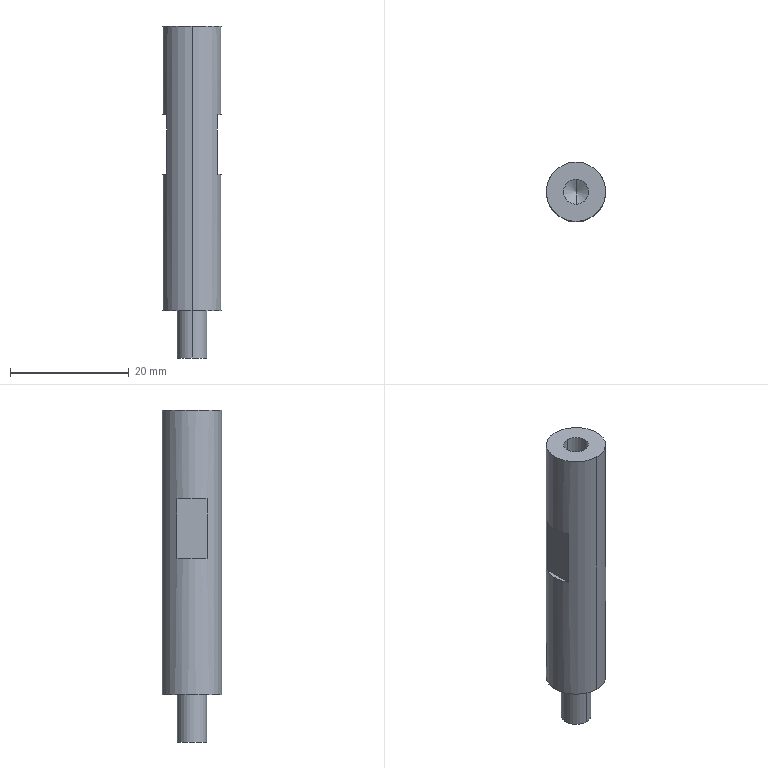Component | SolidWorks | YS01-059CylinderExtensionRod-2 | 1 solid | 17 faces | box 10 x 10 x 56 mm | volume 3701 mm3 | plane 9 | cylinder 6 | cone 2 | commonest cylinder face diameters 5 x2 4.2 x2 10 x2
build123d program:
from build123d import *

# Parameters (mm, degrees)
SKETCH1_R             = 5
BOSS_EXTRUDE1_DEPTH   = 48
M5_TAPPED_HOLE1_D     = 4.2
M5_TAPPED_HOLE1_DEPTH = 12.4
M5_TAPPED_HOLE1_TIP   = 1.262
SKETCH4_R             = 2.5
BOSS_EXTRUDE2_DEPTH   = 8
SKETCH5_W             = 15.912
SKETCH5_H             = 5.844
SKETCH5_H_2           = 6.454
CUT_EXTRUDE1_DEPTH    = 10


with BuildPart() as part:
    # Sketch1 → Boss-Extrude1 (new body)
    with BuildSketch(Plane.XY):
        Circle(SKETCH1_R)
    extrude(amount=BOSS_EXTRUDE1_DEPTH)

    # M5 Tapped Hole1
    with Locations(Plane.XY.offset(48)):
        with Locations((0, 0)):
            Hole(M5_TAPPED_HOLE1_D / 2, depth=M5_TAPPED_HOLE1_DEPTH)
            with Locations((0, 0, -(M5_TAPPED_HOLE1_DEPTH + M5_TAPPED_HOLE1_TIP / 2))):  # 118° drill point
                Cone(0, M5_TAPPED_HOLE1_D / 2, M5_TAPPED_HOLE1_TIP, mode=Mode.SUBTRACT)

    # Sketch4 → Boss-Extrude2 (add)
    with BuildSketch(Plane(origin=(0, 0, 0), x_dir=(-1, 0, 0), z_dir=(0, 0, -1))):
        with Locations(Location((0, 0, 0), (0, 0, 180))):
            Circle(SKETCH4_R)
    extrude(amount=BOSS_EXTRUDE2_DEPTH)

    # Sketch5 → Cut-Extrude1 (cut)
    with BuildSketch(Plane.XY.offset(33)):
        with Locations((1.405, 7.222)):
            Rectangle(SKETCH5_W, SKETCH5_H)
        with Locations((1.405, -7.527)):
            Rectangle(SKETCH5_W, SKETCH5_H_2)
    extrude(amount=-CUT_EXTRUDE1_DEPTH, mode=Mode.SUBTRACT)


solid = part.part

# Placed as in the assembly
solid = solid.moved(Location((-566.612, -123.873, 2470.4), (0, 0, 90)))
STEP:
#1=CARTESIAN_POINT('',(-22.308,-4.975,96.945));
#2=VERTEX_POINT('',#1);
#3=CARTESIAN_POINT('',(-22.308,-4.778,96.945));
#4=VERTEX_POINT('',#3);
#5=CARTESIAN_POINT('',(-22.308,-4.877,96.945));
#6=DIRECTION('',(0.,0.,-1.));
#7=DIRECTION('',(0.,-1.,0.));
#8=AXIS2_PLACEMENT_3D('',#5,#6,#7);
#9=CIRCLE('',#8,0.09843);
#10=EDGE_CURVE('',#2,#4,#9,.T.);
#11=ORIENTED_EDGE('',*,*,#10,.F.);
#12=CARTESIAN_POINT('',(-22.308,-4.975,97.26));
#13=VERTEX_POINT('',#12);
#14=CARTESIAN_POINT('',(-22.308,-4.975,96.945));
#15=DIRECTION('',(0.,0.,1.));
#16=VECTOR('',#15,39.37);
#17=LINE('',#14,#16);
#18=EDGE_CURVE('',#2,#13,#17,.T.);
#19=ORIENTED_EDGE('',*,*,#18,.T.);
#20=CARTESIAN_POINT('',(-22.308,-4.778,97.26));
#21=VERTEX_POINT('',#20);
#22=CARTESIAN_POINT('',(-22.308,-4.877,97.26));
#23=DIRECTION('',(0.,0.,-1.));
#24=DIRECTION('',(0.,1.,0.));
#25=AXIS2_PLACEMENT_3D('',#22,#23,#24);
#26=CIRCLE('',#25,0.09843);
#27=EDGE_CURVE('',#13,#21,#26,.T.);
#28=ORIENTED_EDGE('',*,*,#27,.T.);
#29=CARTESIAN_POINT('',(-22.308,-4.778,96.945));
#30=DIRECTION('',(0.,0.,1.));
#31=VECTOR('',#30,39.37);
#32=LINE('',#29,#31);
#33=EDGE_CURVE('',#4,#21,#32,.T.);
#34=ORIENTED_EDGE('',*,*,#33,.F.);
#35=EDGE_LOOP('',(#11,#19,#28,#34));
#36=FACE_OUTER_BOUND('',#35,.T.);
#37=CARTESIAN_POINT('',(-22.308,-4.877,96.945));
#38=DIRECTION('',(0.,0.,1.));
#39=DIRECTION('',(0.,1.,0.));
#40=AXIS2_PLACEMENT_3D('',#37,#38,#39);
#41=CYLINDRICAL_SURFACE('',#40,0.09843);
#42=ADVANCED_FACE('',(#36),#41,.T.);
#43=CARTESIAN_POINT('',(-22.308,-4.96,98.661));
#44=VERTEX_POINT('',#43);
#45=CARTESIAN_POINT('',(-22.308,-4.794,98.661));
#46=VERTEX_POINT('',#45);
#47=CARTESIAN_POINT('',(-22.308,-4.877,98.661));
#48=DIRECTION('',(0.,0.,1.));
#49=DIRECTION('',(0.,1.,0.));
#50=AXIS2_PLACEMENT_3D('',#47,#48,#49);
#51=CIRCLE('',#50,0.08268);
#52=EDGE_CURVE('',#44,#46,#51,.T.);
#53=ORIENTED_EDGE('',*,*,#52,.F.);
#54=CARTESIAN_POINT('',(-22.308,-4.96,99.15));
#55=VERTEX_POINT('',#54);
#56=CARTESIAN_POINT('',(-22.308,-4.96,99.15));
#57=DIRECTION('',(0.,0.,1.));
#58=VECTOR('',#57,39.37);
#59=LINE('',#56,#58);
#60=EDGE_CURVE('',#44,#55,#59,.T.);
#61=ORIENTED_EDGE('',*,*,#60,.T.);
#62=CARTESIAN_POINT('',(-22.308,-4.794,99.15));
#63=VERTEX_POINT('',#62);
#64=CARTESIAN_POINT('',(-22.308,-4.877,99.15));
#65=DIRECTION('',(0.,0.,1.));
#66=DIRECTION('',(0.,1.,0.));
#67=AXIS2_PLACEMENT_3D('',#64,#65,#66);
#68=CIRCLE('',#67,0.08268);
#69=EDGE_CURVE('',#55,#63,#68,.T.);
#70=ORIENTED_EDGE('',*,*,#69,.T.);
#71=CARTESIAN_POINT('',(-22.308,-4.794,99.15));
#72=DIRECTION('',(0.,0.,1.));
#73=VECTOR('',#72,39.37);
#74=LINE('',#71,#73);
#75=EDGE_CURVE('',#46,#63,#74,.T.);
#76=ORIENTED_EDGE('',*,*,#75,.F.);
#77=EDGE_LOOP('',(#53,#61,#70,#76));
#78=FACE_OUTER_BOUND('',#77,.T.);
#79=CARTESIAN_POINT('',(-22.308,-4.877,99.15));
#80=DIRECTION('',(0.,0.,1.));
#81=DIRECTION('',(0.,1.,0.));
#82=AXIS2_PLACEMENT_3D('',#79,#80,#81);
#83=CYLINDRICAL_SURFACE('',#82,0.08268);
#84=ADVANCED_FACE('',(#78),#83,.F.);
#85=CARTESIAN_POINT('',(-22.308,-4.877,98.612));
#86=VERTEX_POINT('',#85);
#87=CARTESIAN_POINT('',(-22.308,-4.794,98.661));
#88=DIRECTION('',(-0.,0.8572,0.515));
#89=VECTOR('',#88,39.37);
#90=LINE('',#87,#89);
#91=EDGE_CURVE('',#86,#46,#90,.T.);
#92=ORIENTED_EDGE('',*,*,#91,.F.);
#93=CARTESIAN_POINT('',(-22.308,-4.96,98.661));
#94=DIRECTION('',(0.,-0.8572,0.515));
#95=VECTOR('',#94,39.37);
#96=LINE('',#93,#95);
#97=EDGE_CURVE('',#86,#44,#96,.T.);
#98=ORIENTED_EDGE('',*,*,#97,.T.);
#99=ORIENTED_EDGE('',*,*,#52,.T.);
#100=EDGE_LOOP('',(#92,#98,#99));
#101=FACE_OUTER_BOUND('',#100,.T.);
#102=CARTESIAN_POINT('',(-22.308,-4.877,98.661));
#103=DIRECTION('',(0.,0.,1.));
#104=DIRECTION('',(0.,1.,0.));
#105=AXIS2_PLACEMENT_3D('',#102,#103,#104);
#106=CONICAL_SURFACE('',#105,0.08268,1.03);
#107=ADVANCED_FACE('',(#101),#106,.F.);
#108=CARTESIAN_POINT('',(-22.477,-4.776,98.165));
#109=VERTEX_POINT('',#108);
#110=CARTESIAN_POINT('',(-22.477,-4.977,98.165));
#111=VERTEX_POINT('',#110);
#112=CARTESIAN_POINT('',(-22.308,-4.877,98.165));
#113=DIRECTION('',(0.,0.,1.));
#114=DIRECTION('',(0.,1.,0.));
#115=AXIS2_PLACEMENT_3D('',#112,#113,#114);
#116=CIRCLE('',#115,0.1969);
#117=EDGE_CURVE('',#109,#111,#116,.T.);
#118=ORIENTED_EDGE('',*,*,#117,.F.);
#119=CARTESIAN_POINT('',(-22.477,-4.776,98.559));
#120=VERTEX_POINT('',#119);
#121=CARTESIAN_POINT('',(-22.477,-4.776,99.15));
#122=DIRECTION('',(0.,0.,1.));
#123=VECTOR('',#122,39.37);
#124=LINE('',#121,#123);
#125=EDGE_CURVE('',#109,#120,#124,.T.);
#126=ORIENTED_EDGE('',*,*,#125,.T.);
#127=CARTESIAN_POINT('',(-22.477,-4.977,98.559));
#128=VERTEX_POINT('',#127);
#129=CARTESIAN_POINT('',(-22.308,-4.877,98.559));
#130=DIRECTION('',(0.,0.,1.));
#131=DIRECTION('',(0.,1.,0.));
#132=AXIS2_PLACEMENT_3D('',#129,#130,#131);
#133=CIRCLE('',#132,0.1969);
#134=EDGE_CURVE('',#120,#128,#133,.T.);
#135=ORIENTED_EDGE('',*,*,#134,.T.);
#136=CARTESIAN_POINT('',(-22.477,-4.977,99.15));
#137=DIRECTION('',(0.,0.,-1.));
#138=VECTOR('',#137,39.37);
#139=LINE('',#136,#138);
#140=EDGE_CURVE('',#128,#111,#139,.T.);
#141=ORIENTED_EDGE('',*,*,#140,.T.);
#142=EDGE_LOOP('',(#118,#126,#135,#141));
#143=FACE_BOUND('',#142,.T.);
#144=CARTESIAN_POINT('',(-22.308,-4.68,99.15));
#145=VERTEX_POINT('',#144);
#146=CARTESIAN_POINT('',(-22.308,-5.074,99.15));
#147=VERTEX_POINT('',#146);
#148=CARTESIAN_POINT('',(-22.308,-4.877,99.15));
#149=DIRECTION('',(0.,0.,1.));
#150=DIRECTION('',(0.,1.,0.));
#151=AXIS2_PLACEMENT_3D('',#148,#149,#150);
#152=CIRCLE('',#151,0.1969);
#153=EDGE_CURVE('',#145,#147,#152,.T.);
#154=ORIENTED_EDGE('',*,*,#153,.F.);
#155=CARTESIAN_POINT('',(-22.308,-4.68,97.26));
#156=VERTEX_POINT('',#155);
#157=CARTESIAN_POINT('',(-22.308,-4.68,99.15));
#158=DIRECTION('',(0.,0.,-1.));
#159=VECTOR('',#158,39.37);
#160=LINE('',#157,#159);
#161=EDGE_CURVE('',#145,#156,#160,.T.);
#162=ORIENTED_EDGE('',*,*,#161,.T.);
#163=CARTESIAN_POINT('',(-22.308,-5.074,97.26));
#164=VERTEX_POINT('',#163);
#165=CARTESIAN_POINT('',(-22.308,-4.877,97.26));
#166=DIRECTION('',(0.,0.,1.));
#167=DIRECTION('',(0.,1.,0.));
#168=AXIS2_PLACEMENT_3D('',#165,#166,#167);
#169=CIRCLE('',#168,0.1969);
#170=EDGE_CURVE('',#156,#164,#169,.T.);
#171=ORIENTED_EDGE('',*,*,#170,.T.);
#172=CARTESIAN_POINT('',(-22.308,-5.074,99.15));
#173=DIRECTION('',(0.,0.,-1.));
#174=VECTOR('',#173,39.37);
#175=LINE('',#172,#174);
#176=EDGE_CURVE('',#147,#164,#175,.T.);
#177=ORIENTED_EDGE('',*,*,#176,.F.);
#178=EDGE_LOOP('',(#154,#162,#171,#177));
#179=FACE_OUTER_BOUND('',#178,.T.);
#180=CARTESIAN_POINT('',(-22.308,-4.877,99.15));
#181=DIRECTION('',(0.,0.,-1.));
#182=DIRECTION('',(0.,-1.,0.));
#183=AXIS2_PLACEMENT_3D('',#180,#181,#182);
#184=CYLINDRICAL_SURFACE('',#183,0.1969);
#185=ADVANCED_FACE('',(#143,#179),#184,.T.);
#186=ORIENTED_EDGE('',*,*,#161,.F.);
#187=CARTESIAN_POINT('',(-22.308,-4.877,99.15));
#188=DIRECTION('',(0.,0.,1.));
#189=DIRECTION('',(0.,1.,0.));
#190=AXIS2_PLACEMENT_3D('',#187,#188,#189);
#191=CIRCLE('',#190,0.1969);
#192=EDGE_CURVE('',#147,#145,#191,.T.);
#193=ORIENTED_EDGE('',*,*,#192,.F.);
#194=ORIENTED_EDGE('',*,*,#176,.T.);
#195=CARTESIAN_POINT('',(-22.308,-4.877,97.26));
#196=DIRECTION('',(0.,0.,1.));
#197=DIRECTION('',(0.,1.,0.));
#198=AXIS2_PLACEMENT_3D('',#195,#196,#197);
#199=CIRCLE('',#198,0.1969);
#200=EDGE_CURVE('',#164,#156,#199,.T.);
#201=ORIENTED_EDGE('',*,*,#200,.T.);
#202=EDGE_LOOP('',(#186,#193,#194,#201));
#203=FACE_OUTER_BOUND('',#202,.T.);
#204=CARTESIAN_POINT('',(-22.138,-4.977,98.165));
#205=VERTEX_POINT('',#204);
#206=CARTESIAN_POINT('',(-22.138,-4.776,98.165));
#207=VERTEX_POINT('',#206);
#208=CARTESIAN_POINT('',(-22.308,-4.877,98.165));
#209=DIRECTION('',(0.,0.,1.));
#210=DIRECTION('',(0.,1.,0.));
#211=AXIS2_PLACEMENT_3D('',#208,#209,#210);
#212=CIRCLE('',#211,0.1969);
#213=EDGE_CURVE('',#205,#207,#212,.T.);
#214=ORIENTED_EDGE('',*,*,#213,.F.);
#215=CARTESIAN_POINT('',(-22.138,-4.977,98.559));
#216=VERTEX_POINT('',#215);
#217=CARTESIAN_POINT('',(-22.138,-4.977,99.15));
#218=DIRECTION('',(0.,0.,1.));
#219=VECTOR('',#218,39.37);
#220=LINE('',#217,#219);
#221=EDGE_CURVE('',#205,#216,#220,.T.);
#222=ORIENTED_EDGE('',*,*,#221,.T.);
#223=CARTESIAN_POINT('',(-22.138,-4.776,98.559));
#224=VERTEX_POINT('',#223);
#225=CARTESIAN_POINT('',(-22.308,-4.877,98.559));
#226=DIRECTION('',(0.,0.,1.));
#227=DIRECTION('',(0.,1.,0.));
#228=AXIS2_PLACEMENT_3D('',#225,#226,#227);
#229=CIRCLE('',#228,0.1969);
#230=EDGE_CURVE('',#216,#224,#229,.T.);
#231=ORIENTED_EDGE('',*,*,#230,.T.);
#232=CARTESIAN_POINT('',(-22.138,-4.776,99.15));
#233=DIRECTION('',(0.,0.,-1.));
#234=VECTOR('',#233,39.37);
#235=LINE('',#232,#234);
#236=EDGE_CURVE('',#224,#207,#235,.T.);
#237=ORIENTED_EDGE('',*,*,#236,.T.);
#238=EDGE_LOOP('',(#214,#222,#231,#237));
#239=FACE_BOUND('',#238,.T.);
#240=CARTESIAN_POINT('',(-22.308,-4.877,99.15));
#241=DIRECTION('',(0.,0.,-1.));
#242=DIRECTION('',(0.,-1.,0.));
#243=AXIS2_PLACEMENT_3D('',#240,#241,#242);
#244=CYLINDRICAL_SURFACE('',#243,0.1969);
#245=ADVANCED_FACE('',(#203,#239),#244,.T.);
#246=ORIENTED_EDGE('',*,*,#200,.F.);
#247=ORIENTED_EDGE('',*,*,#170,.F.);
#248=EDGE_LOOP('',(#246,#247));
#249=FACE_OUTER_BOUND('',#248,.T.);
#250=CARTESIAN_POINT('',(-22.308,-4.877,97.26));
#251=DIRECTION('',(0.,0.,-1.));
#252=DIRECTION('',(0.,1.,0.));
#253=AXIS2_PLACEMENT_3D('',#250,#251,#252);
#254=CIRCLE('',#253,0.09843);
#255=EDGE_CURVE('',#21,#13,#254,.T.);
#256=ORIENTED_EDGE('',*,*,#255,.F.);
#257=ORIENTED_EDGE('',*,*,#27,.F.);
#258=EDGE_LOOP('',(#256,#257));
#259=FACE_BOUND('',#258,.T.);
#260=CARTESIAN_POINT('',(-22.308,-4.877,97.26));
#261=DIRECTION('',(0.,0.,1.));
#262=DIRECTION('',(-0.,1.,0.));
#263=AXIS2_PLACEMENT_3D('',#260,#261,#262);
#264=PLANE('',#263);
#265=ADVANCED_FACE('',(#249,#259),#264,.F.);
#266=CARTESIAN_POINT('',(-22.308,-4.877,99.15));
#267=DIRECTION('',(0.,0.,1.));
#268=DIRECTION('',(0.,1.,0.));
#269=AXIS2_PLACEMENT_3D('',#266,#267,#268);
#270=CIRCLE('',#269,0.08268);
#271=EDGE_CURVE('',#63,#55,#270,.T.);
#272=ORIENTED_EDGE('',*,*,#271,.F.);
#273=ORIENTED_EDGE('',*,*,#69,.F.);
#274=EDGE_LOOP('',(#272,#273));
#275=FACE_BOUND('',#274,.T.);
#276=ORIENTED_EDGE('',*,*,#192,.T.);
#277=ORIENTED_EDGE('',*,*,#153,.T.);
#278=EDGE_LOOP('',(#276,#277));
#279=FACE_OUTER_BOUND('',#278,.T.);
#280=CARTESIAN_POINT('',(-22.308,-4.877,99.15));
#281=DIRECTION('',(0.,0.,1.));
#282=DIRECTION('',(-0.,1.,0.));
#283=AXIS2_PLACEMENT_3D('',#280,#281,#282);
#284=PLANE('',#283);
#285=ADVANCED_FACE('',(#275,#279),#284,.T.);
#286=ORIENTED_EDGE('',*,*,#97,.F.);
#287=ORIENTED_EDGE('',*,*,#91,.T.);
#288=CARTESIAN_POINT('',(-22.308,-4.877,98.661));
#289=DIRECTION('',(0.,0.,1.));
#290=DIRECTION('',(0.,1.,0.));
#291=AXIS2_PLACEMENT_3D('',#288,#289,#290);
#292=CIRCLE('',#291,0.08268);
#293=EDGE_CURVE('',#46,#44,#292,.T.);
#294=ORIENTED_EDGE('',*,*,#293,.T.);
#295=EDGE_LOOP('',(#286,#287,#294));
#296=FACE_OUTER_BOUND('',#295,.T.);
#297=CARTESIAN_POINT('',(-22.308,-4.877,98.661));
#298=DIRECTION('',(0.,0.,1.));
#299=DIRECTION('',(0.,1.,0.));
#300=AXIS2_PLACEMENT_3D('',#297,#298,#299);
#301=CONICAL_SURFACE('',#300,0.08268,1.03);
#302=ADVANCED_FACE('',(#296),#301,.F.);
#303=ORIENTED_EDGE('',*,*,#60,.F.);
#304=ORIENTED_EDGE('',*,*,#293,.F.);
#305=ORIENTED_EDGE('',*,*,#75,.T.);
#306=ORIENTED_EDGE('',*,*,#271,.T.);
#307=EDGE_LOOP('',(#303,#304,#305,#306));
#308=FACE_OUTER_BOUND('',#307,.T.);
#309=CARTESIAN_POINT('',(-22.308,-4.877,99.15));
#310=DIRECTION('',(0.,0.,1.));
#311=DIRECTION('',(0.,1.,0.));
#312=AXIS2_PLACEMENT_3D('',#309,#310,#311);
#313=CYLINDRICAL_SURFACE('',#312,0.08268);
#314=ADVANCED_FACE('',(#308),#313,.F.);
#315=ORIENTED_EDGE('',*,*,#18,.F.);
#316=CARTESIAN_POINT('',(-22.308,-4.877,96.945));
#317=DIRECTION('',(0.,0.,-1.));
#318=DIRECTION('',(0.,-1.,0.));
#319=AXIS2_PLACEMENT_3D('',#316,#317,#318);
#320=CIRCLE('',#319,0.09843);
#321=EDGE_CURVE('',#4,#2,#320,.T.);
#322=ORIENTED_EDGE('',*,*,#321,.F.);
#323=ORIENTED_EDGE('',*,*,#33,.T.);
#324=ORIENTED_EDGE('',*,*,#255,.T.);
#325=EDGE_LOOP('',(#315,#322,#323,#324));
#326=FACE_OUTER_BOUND('',#325,.T.);
#327=CARTESIAN_POINT('',(-22.308,-4.877,96.945));
#328=DIRECTION('',(0.,0.,1.));
#329=DIRECTION('',(0.,1.,0.));
#330=AXIS2_PLACEMENT_3D('',#327,#328,#329);
#331=CYLINDRICAL_SURFACE('',#330,0.09843);
#332=ADVANCED_FACE('',(#326),#331,.T.);
#333=ORIENTED_EDGE('',*,*,#321,.T.);
#334=ORIENTED_EDGE('',*,*,#10,.T.);
#335=EDGE_LOOP('',(#333,#334));
#336=FACE_OUTER_BOUND('',#335,.T.);
#337=CARTESIAN_POINT('',(-22.308,-4.877,96.945));
#338=DIRECTION('',(0.,0.,-1.));
#339=DIRECTION('',(0.,-1.,0.));
#340=AXIS2_PLACEMENT_3D('',#337,#338,#339);
#341=PLANE('',#340);
#342=ADVANCED_FACE('',(#336),#341,.T.);
#343=CARTESIAN_POINT('',(-22.477,-5.135,98.559));
#344=DIRECTION('',(-0.,1.,0.));
#345=VECTOR('',#344,39.37);
#346=LINE('',#343,#345);
#347=EDGE_CURVE('',#128,#120,#346,.T.);
#348=ORIENTED_EDGE('',*,*,#347,.T.);
#349=ORIENTED_EDGE('',*,*,#125,.F.);
#350=CARTESIAN_POINT('',(-22.477,-5.135,98.165));
#351=DIRECTION('',(-0.,1.,0.));
#352=VECTOR('',#351,39.37);
#353=LINE('',#350,#352);
#354=EDGE_CURVE('',#111,#109,#353,.T.);
#355=ORIENTED_EDGE('',*,*,#354,.F.);
#356=ORIENTED_EDGE('',*,*,#140,.F.);
#357=EDGE_LOOP('',(#348,#349,#355,#356));
#358=FACE_OUTER_BOUND('',#357,.T.);
#359=CARTESIAN_POINT('',(-22.477,-5.135,98.165));
#360=DIRECTION('',(1.,0.,0.));
#361=DIRECTION('',(0.,0.,-1.));
#362=AXIS2_PLACEMENT_3D('',#359,#360,#361);
#363=PLANE('',#362);
#364=ADVANCED_FACE('',(#358),#363,.F.);
#365=ORIENTED_EDGE('',*,*,#117,.T.);
#366=ORIENTED_EDGE('',*,*,#354,.T.);
#367=EDGE_LOOP('',(#365,#366));
#368=FACE_OUTER_BOUND('',#367,.T.);
#369=CARTESIAN_POINT('',(-22.308,-4.877,98.165));
#370=DIRECTION('',(0.,0.,1.));
#371=DIRECTION('',(-0.,1.,0.));
#372=AXIS2_PLACEMENT_3D('',#369,#370,#371);
#373=PLANE('',#372);
#374=ADVANCED_FACE('',(#368),#373,.T.);
#375=ORIENTED_EDGE('',*,*,#347,.F.);
#376=ORIENTED_EDGE('',*,*,#134,.F.);
#377=EDGE_LOOP('',(#375,#376));
#378=FACE_OUTER_BOUND('',#377,.T.);
#379=CARTESIAN_POINT('',(-22.308,-4.877,98.559));
#380=DIRECTION('',(0.,0.,1.));
#381=DIRECTION('',(-0.,1.,0.));
#382=AXIS2_PLACEMENT_3D('',#379,#380,#381);
#383=PLANE('',#382);
#384=ADVANCED_FACE('',(#378),#383,.F.);
#385=CARTESIAN_POINT('',(-22.138,-5.135,98.559));
#386=DIRECTION('',(0.,-1.,0.));
#387=VECTOR('',#386,39.37);
#388=LINE('',#385,#387);
#389=EDGE_CURVE('',#224,#216,#388,.T.);
#390=ORIENTED_EDGE('',*,*,#389,.T.);
#391=ORIENTED_EDGE('',*,*,#221,.F.);
#392=CARTESIAN_POINT('',(-22.138,-5.135,98.165));
#393=DIRECTION('',(0.,-1.,0.));
#394=VECTOR('',#393,39.37);
#395=LINE('',#392,#394);
#396=EDGE_CURVE('',#207,#205,#395,.T.);
#397=ORIENTED_EDGE('',*,*,#396,.F.);
#398=ORIENTED_EDGE('',*,*,#236,.F.);
#399=EDGE_LOOP('',(#390,#391,#397,#398));
#400=FACE_OUTER_BOUND('',#399,.T.);
#401=CARTESIAN_POINT('',(-22.138,-5.135,98.165));
#402=DIRECTION('',(-1.,-0.,0.));
#403=DIRECTION('',(0.,0.,1.));
#404=AXIS2_PLACEMENT_3D('',#401,#402,#403);
#405=PLANE('',#404);
#406=ADVANCED_FACE('',(#400),#405,.F.);
#407=ORIENTED_EDGE('',*,*,#213,.T.);
#408=ORIENTED_EDGE('',*,*,#396,.T.);
#409=EDGE_LOOP('',(#407,#408));
#410=FACE_OUTER_BOUND('',#409,.T.);
#411=CARTESIAN_POINT('',(-22.308,-4.877,98.165));
#412=DIRECTION('',(0.,0.,1.));
#413=DIRECTION('',(-0.,1.,0.));
#414=AXIS2_PLACEMENT_3D('',#411,#412,#413);
#415=PLANE('',#414);
#416=ADVANCED_FACE('',(#410),#415,.T.);
#417=ORIENTED_EDGE('',*,*,#389,.F.);
#418=ORIENTED_EDGE('',*,*,#230,.F.);
#419=EDGE_LOOP('',(#417,#418));
#420=FACE_OUTER_BOUND('',#419,.T.);
#421=CARTESIAN_POINT('',(-22.308,-4.877,98.559));
#422=DIRECTION('',(0.,0.,1.));
#423=DIRECTION('',(-0.,1.,0.));
#424=AXIS2_PLACEMENT_3D('',#421,#422,#423);
#425=PLANE('',#424);
#426=ADVANCED_FACE('',(#420),#425,.F.);
#427=CLOSED_SHELL('',(#42,#84,#107,#185,#245,#265,#285,#302,#314,#332,#342,#364,#374,#384,#406,#416,#426));
#428=MANIFOLD_SOLID_BREP('',#427);
#429=CARTESIAN_POINT('',(0.,0.,0.));
#430=DIRECTION('',(0.,0.,1.));
#431=DIRECTION('',(1.,0.,0.));
#432=AXIS2_PLACEMENT_3D('',#429,#430,#431);
#433=(LENGTH_UNIT()NAMED_UNIT(*)SI_UNIT($,.METRE.));
#434=LENGTH_MEASURE_WITH_UNIT(LENGTH_MEASURE(0.0254),#433);
#435=DIMENSIONAL_EXPONENTS(1.,0.,0.,0.,0.,0.,0.);
#436=(CONVERSION_BASED_UNIT('',#434)LENGTH_UNIT()NAMED_UNIT(#435));
#437=UNCERTAINTY_MEASURE_WITH_UNIT(LENGTH_MEASURE(0.00001),#436,'','');
#438=(NAMED_UNIT(*)PLANE_ANGLE_UNIT()SI_UNIT($,.RADIAN.));
#439=(NAMED_UNIT(*)SI_UNIT($,.STERADIAN.)SOLID_ANGLE_UNIT());
#440=(GEOMETRIC_REPRESENTATION_CONTEXT(3)GLOBAL_UNCERTAINTY_ASSIGNED_CONTEXT((#437))GLOBAL_UNIT_ASSIGNED_CONTEXT((#436,#438,#439))REPRESENTATION_CONTEXT('',''));
#441=ADVANCED_BREP_SHAPE_REPRESENTATION('',(#428,#432),#440);
#442=COLOUR_RGB('',0.7922,0.8196,0.9333);
#443=FILL_AREA_STYLE_COLOUR('',#442);
#444=FILL_AREA_STYLE('',(#443));
#445=SURFACE_STYLE_FILL_AREA(#444);
#446=SURFACE_SIDE_STYLE('',(#445));
#447=SURFACE_STYLE_USAGE(.BOTH.,#446);
#448=PRESENTATION_STYLE_ASSIGNMENT((#447));
#449=STYLED_ITEM('',(#448),#428);
#450=(LENGTH_UNIT()NAMED_UNIT(*)SI_UNIT($,.METRE.));
#451=LENGTH_MEASURE_WITH_UNIT(LENGTH_MEASURE(0.0254),#450);
#452=DIMENSIONAL_EXPONENTS(1.,0.,0.,0.,0.,0.,0.);
#453=(CONVERSION_BASED_UNIT('',#451)LENGTH_UNIT()NAMED_UNIT(#452));
#454=UNCERTAINTY_MEASURE_WITH_UNIT(LENGTH_MEASURE(0.00001),#453,'','');
#455=(NAMED_UNIT(*)PLANE_ANGLE_UNIT()SI_UNIT($,.RADIAN.));
#456=(NAMED_UNIT(*)SI_UNIT($,.STERADIAN.)SOLID_ANGLE_UNIT());
#457=(GEOMETRIC_REPRESENTATION_CONTEXT(3)GLOBAL_UNCERTAINTY_ASSIGNED_CONTEXT((#454))GLOBAL_UNIT_ASSIGNED_CONTEXT((#453,#455,#456))REPRESENTATION_CONTEXT('',''));
#458=MECHANICAL_DESIGN_GEOMETRIC_PRESENTATION_REPRESENTATION('',(#449),#457);
#459=PRESENTATION_LAYER_ASSIGNMENT('','',(#449));